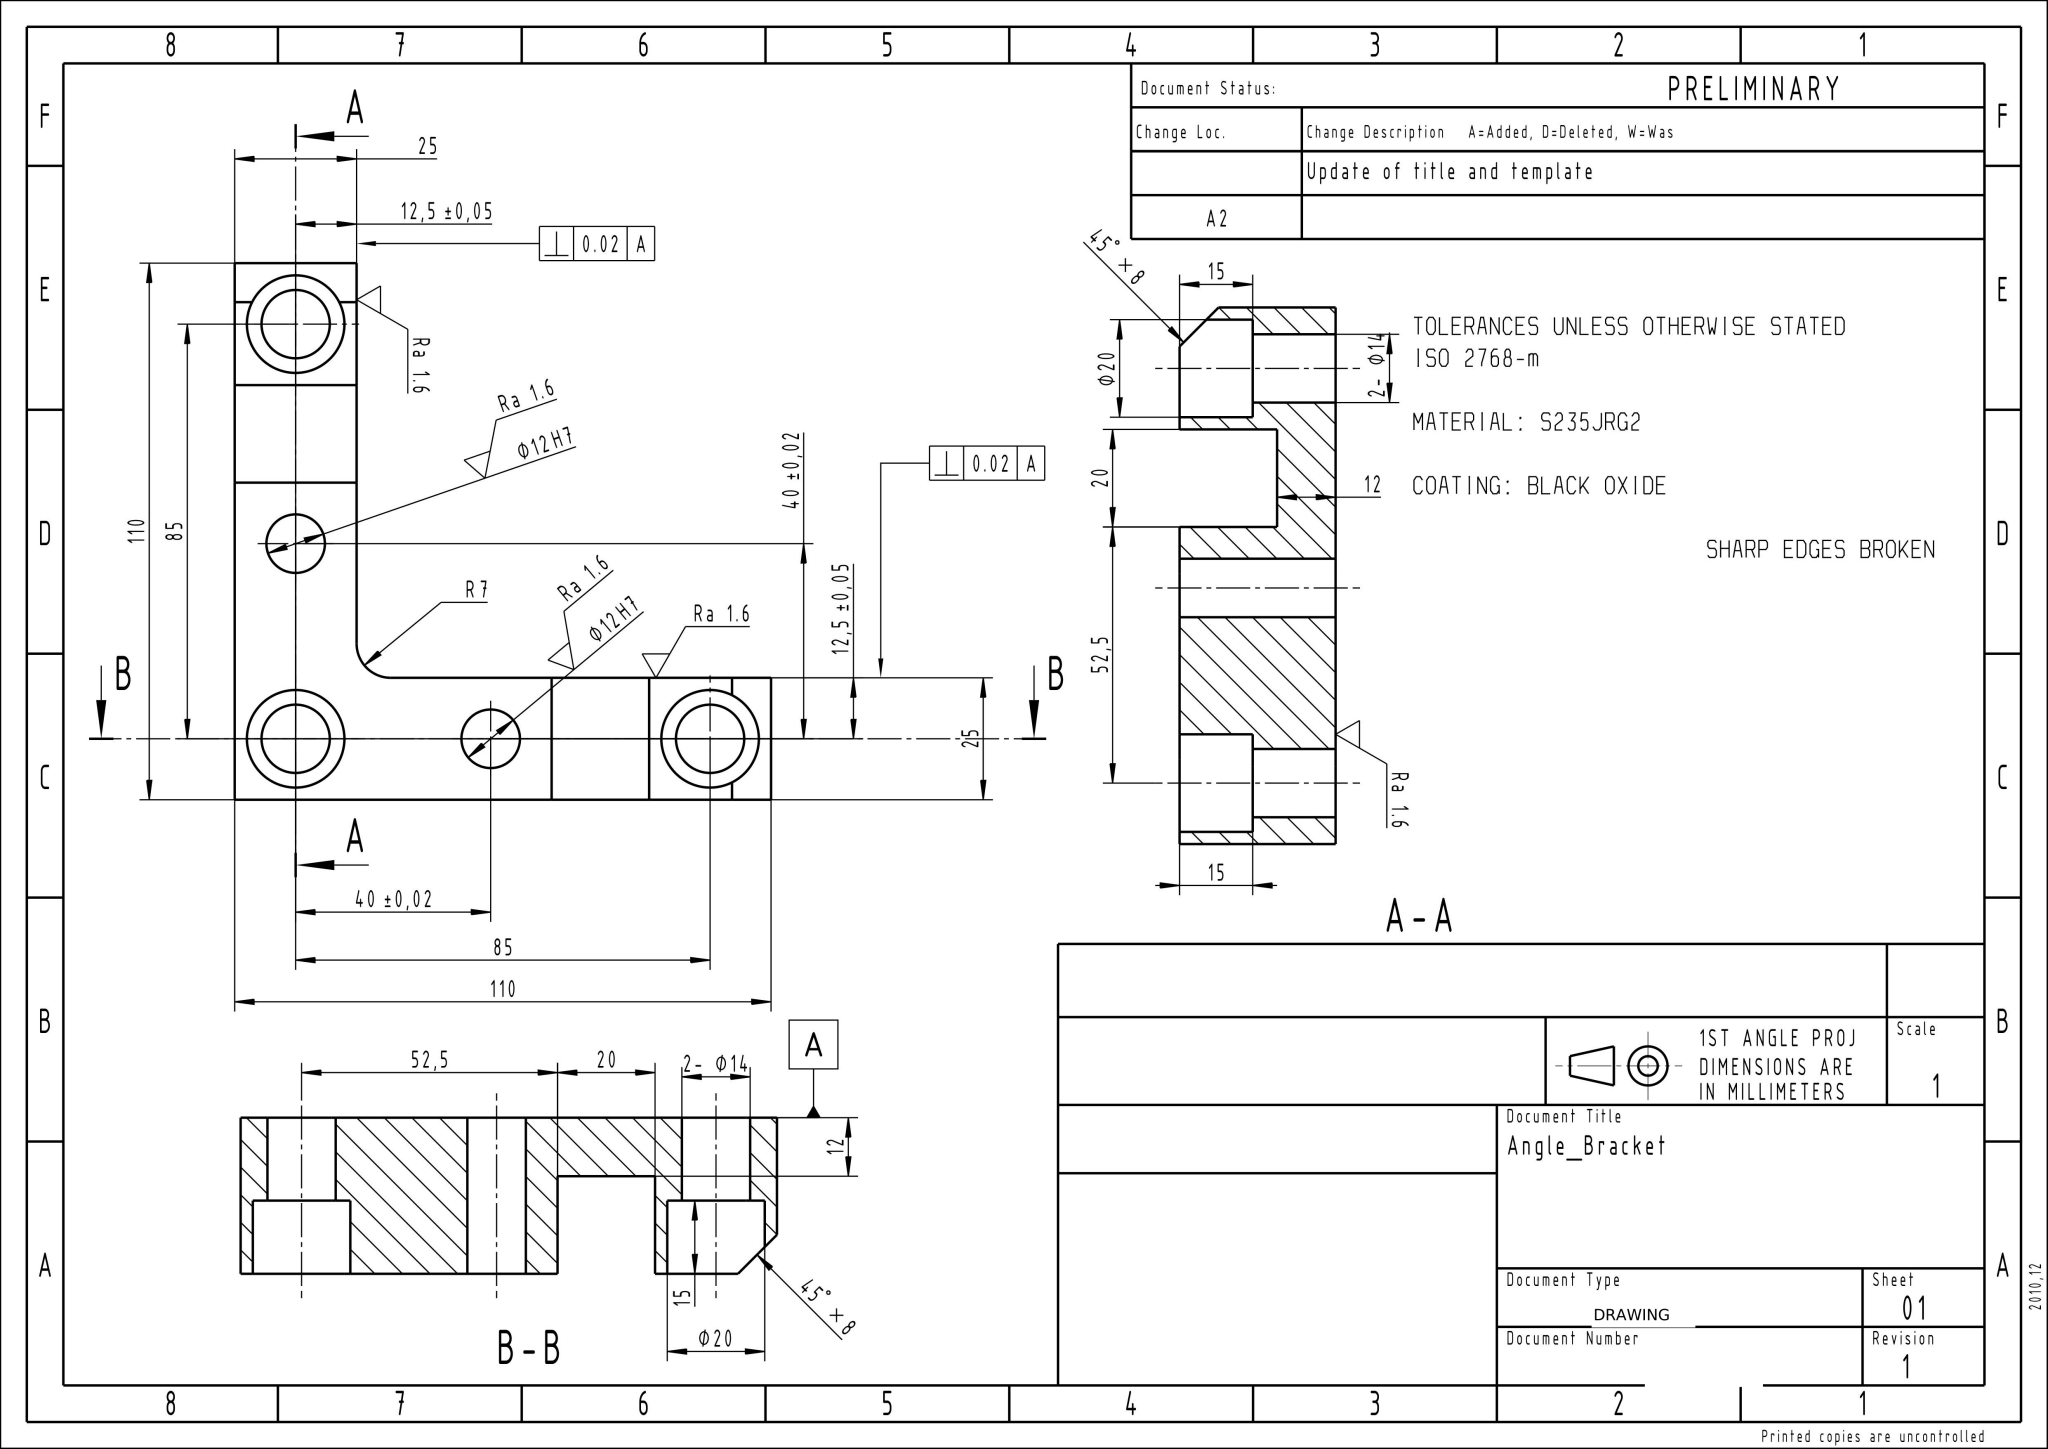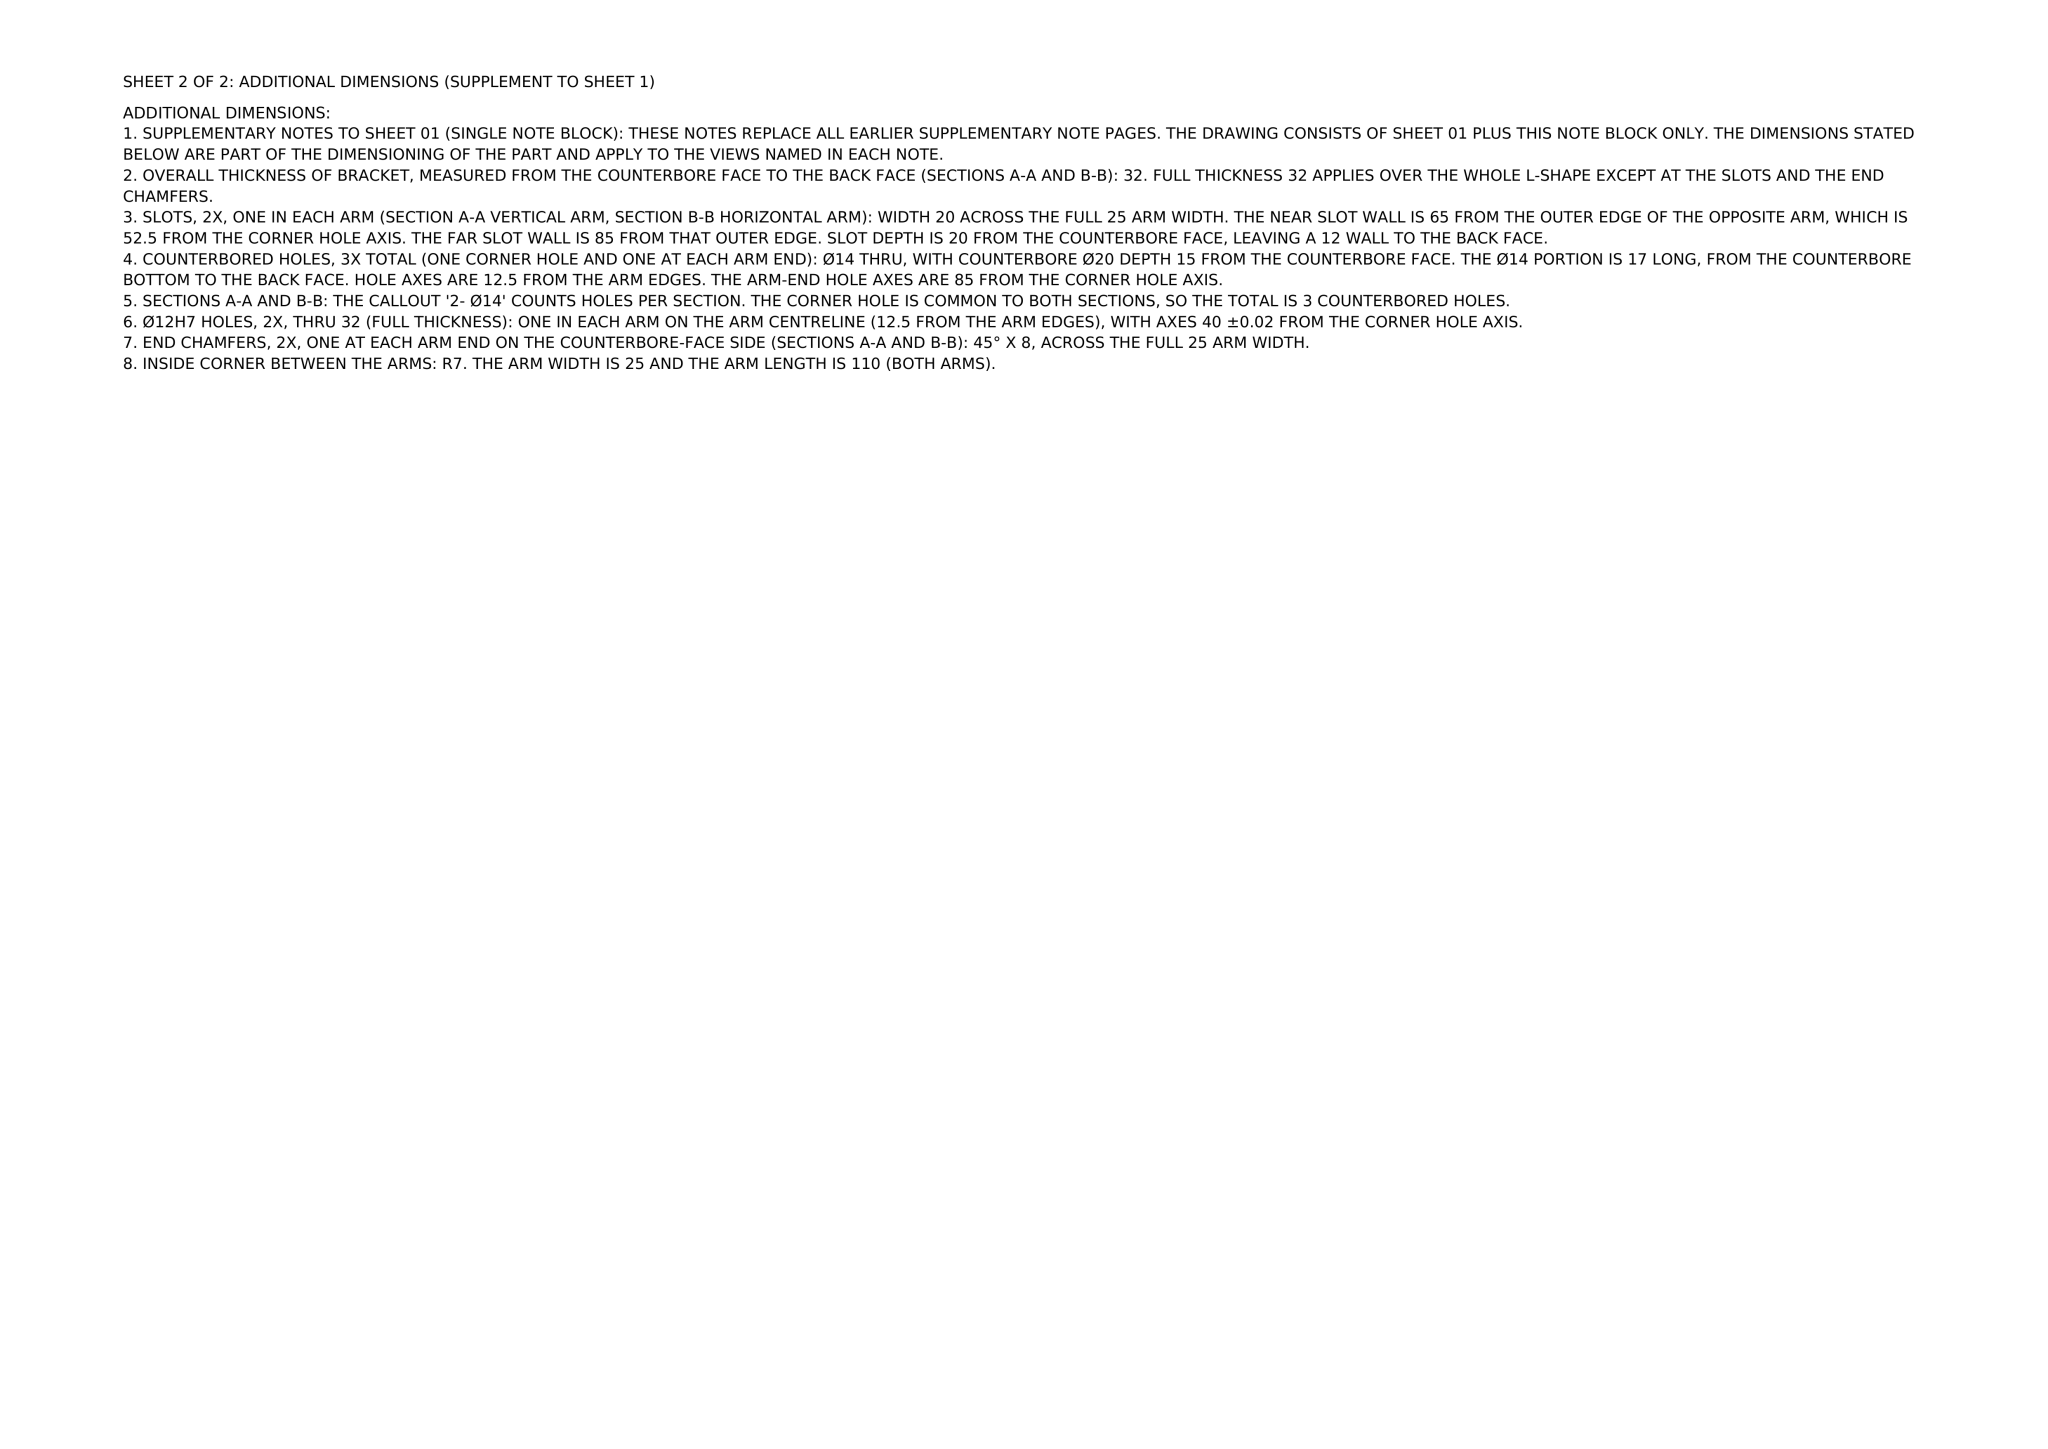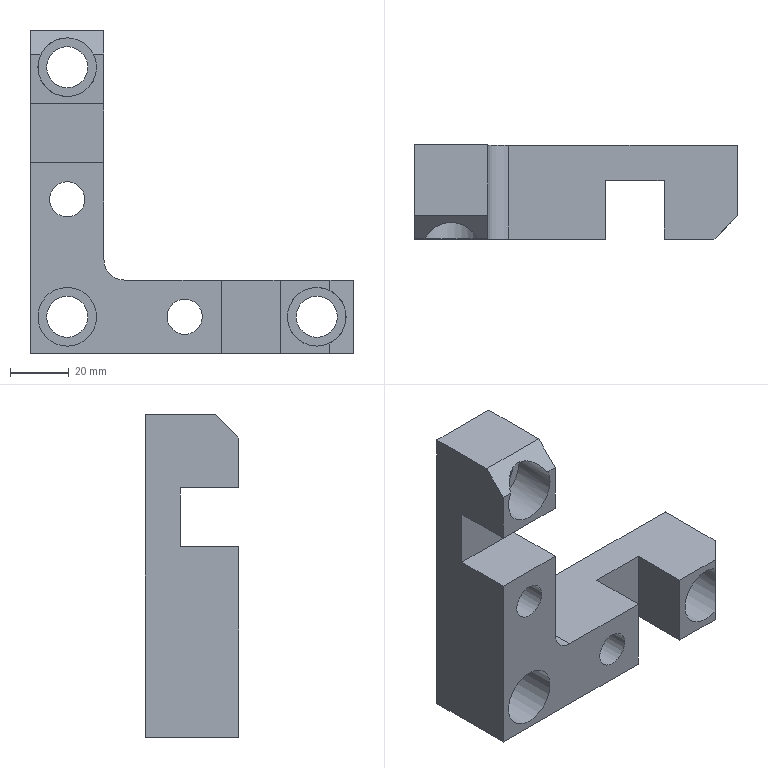Part | NX | mm | 1 solid | 30 faces | box 110 x 32 x 110 mm | volume 105828 mm3 | plane 21 | cylinder 9 | commonest cylinder face diameters 14 x4 20 x3 12 x2
STEP:
#1=CARTESIAN_POINT('',(0.,0.,0.));
#2=DIRECTION('',(0.,0.,1.));
#3=DIRECTION('',(1.,0.,0.));
#4=AXIS2_PLACEMENT_3D('',#1,#2,#3);
#5=(LENGTH_UNIT()NAMED_UNIT(*)SI_UNIT(.MILLI.,.METRE.));
#6=UNCERTAINTY_MEASURE_WITH_UNIT(LENGTH_MEASURE(0.00002),#5,'','');
#7=(NAMED_UNIT(*)PLANE_ANGLE_UNIT()SI_UNIT($,.RADIAN.));
#8=PLANE_ANGLE_MEASURE_WITH_UNIT(PLANE_ANGLE_MEASURE(0.01745),#7);
#9=DIMENSIONAL_EXPONENTS(0.,0.,0.,0.,0.,0.,0.);
#10=(CONVERSION_BASED_UNIT('',#8)NAMED_UNIT(#9)PLANE_ANGLE_UNIT());
#11=(NAMED_UNIT(*)SI_UNIT($,.STERADIAN.)SOLID_ANGLE_UNIT());
#12=(GEOMETRIC_REPRESENTATION_CONTEXT(3)GLOBAL_UNCERTAINTY_ASSIGNED_CONTEXT((#6))GLOBAL_UNIT_ASSIGNED_CONTEXT((#5,#10,#11))REPRESENTATION_CONTEXT('',''));
#13=SHAPE_REPRESENTATION('',(#4),#12);
#14=CARTESIAN_POINT('',(0.,4.,65.));
#15=VERTEX_POINT('',#14);
#16=CARTESIAN_POINT('',(25.,4.,65.));
#17=VERTEX_POINT('',#16);
#18=CARTESIAN_POINT('',(0.,4.,65.));
#19=DIRECTION('',(1.,0.,0.));
#20=VECTOR('',#19,1.);
#21=LINE('',#18,#20);
#22=EDGE_CURVE('',#15,#17,#21,.T.);
#23=ORIENTED_EDGE('',*,*,#22,.F.);
#24=CARTESIAN_POINT('',(0.,-16.,65.));
#25=VERTEX_POINT('',#24);
#26=CARTESIAN_POINT('',(0.,16.,65.));
#27=DIRECTION('',(0.,-1.,0.));
#28=VECTOR('',#27,1.);
#29=LINE('',#26,#28);
#30=EDGE_CURVE('',#15,#25,#29,.T.);
#31=ORIENTED_EDGE('',*,*,#30,.T.);
#32=CARTESIAN_POINT('',(25.,-16.,65.));
#33=VERTEX_POINT('',#32);
#34=CARTESIAN_POINT('',(0.,-16.,65.));
#35=DIRECTION('',(-1.,0.,0.));
#36=VECTOR('',#35,1.);
#37=LINE('',#34,#36);
#38=EDGE_CURVE('',#33,#25,#37,.T.);
#39=ORIENTED_EDGE('',*,*,#38,.F.);
#40=CARTESIAN_POINT('',(25.,16.,65.));
#41=DIRECTION('',(0.,-1.,0.));
#42=VECTOR('',#41,1.);
#43=LINE('',#40,#42);
#44=EDGE_CURVE('',#17,#33,#43,.T.);
#45=ORIENTED_EDGE('',*,*,#44,.F.);
#46=EDGE_LOOP('',(#23,#31,#39,#45));
#47=FACE_OUTER_BOUND('',#46,.T.);
#48=CARTESIAN_POINT('',(32.5,0.,65.));
#49=DIRECTION('',(0.,0.,-1.));
#50=DIRECTION('',(-1.,0.,0.));
#51=AXIS2_PLACEMENT_3D('',#48,#49,#50);
#52=PLANE('',#51);
#53=ADVANCED_FACE('',(#47),#52,.F.);
#54=CARTESIAN_POINT('',(12.5,-1.,19.5));
#55=VERTEX_POINT('',#54);
#56=CARTESIAN_POINT('',(12.5,-1.,12.5));
#57=DIRECTION('',(0.,-1.,0.));
#58=DIRECTION('',(0.,0.,1.));
#59=AXIS2_PLACEMENT_3D('',#56,#57,#58);
#60=CIRCLE('',#59,7.);
#61=EDGE_CURVE('',#55,#55,#60,.T.);
#62=ORIENTED_EDGE('',*,*,#61,.F.);
#63=EDGE_LOOP('',(#62));
#64=FACE_BOUND('',#63,.T.);
#65=CARTESIAN_POINT('',(12.5,-1.,22.5));
#66=VERTEX_POINT('',#65);
#67=CARTESIAN_POINT('',(12.5,-1.,12.5));
#68=DIRECTION('',(0.,-1.,0.));
#69=DIRECTION('',(0.,0.,1.));
#70=AXIS2_PLACEMENT_3D('',#67,#68,#69);
#71=CIRCLE('',#70,10.);
#72=EDGE_CURVE('',#66,#66,#71,.T.);
#73=ORIENTED_EDGE('',*,*,#72,.T.);
#74=EDGE_LOOP('',(#73));
#75=FACE_BOUND('',#74,.T.);
#76=CARTESIAN_POINT('',(12.5,-1.,12.5));
#77=DIRECTION('',(0.,1.,0.));
#78=DIRECTION('',(0.,0.,1.));
#79=AXIS2_PLACEMENT_3D('',#76,#77,#78);
#80=PLANE('',#79);
#81=ADVANCED_FACE('',(#64,#75),#80,.F.);
#82=ORIENTED_EDGE('',*,*,#72,.F.);
#83=EDGE_LOOP('',(#82));
#84=FACE_BOUND('',#83,.T.);
#85=CARTESIAN_POINT('',(12.5,-16.,22.5));
#86=VERTEX_POINT('',#85);
#87=CARTESIAN_POINT('',(12.5,-16.,12.5));
#88=DIRECTION('',(0.,1.,0.));
#89=DIRECTION('',(0.,0.,1.));
#90=AXIS2_PLACEMENT_3D('',#87,#88,#89);
#91=CIRCLE('',#90,10.);
#92=EDGE_CURVE('',#86,#86,#91,.T.);
#93=ORIENTED_EDGE('',*,*,#92,.F.);
#94=EDGE_LOOP('',(#93));
#95=FACE_BOUND('',#94,.T.);
#96=CARTESIAN_POINT('',(12.5,-16.,12.5));
#97=DIRECTION('',(0.,1.,0.));
#98=DIRECTION('',(0.,0.,1.));
#99=AXIS2_PLACEMENT_3D('',#96,#97,#98);
#100=CYLINDRICAL_SURFACE('',#99,10.);
#101=ADVANCED_FACE('',(#84,#95),#100,.F.);
#102=CARTESIAN_POINT('',(110.,16.,0.));
#103=VERTEX_POINT('',#102);
#104=CARTESIAN_POINT('',(110.,-8.,0.));
#105=VERTEX_POINT('',#104);
#106=CARTESIAN_POINT('',(110.,16.,0.));
#107=DIRECTION('',(0.,-1.,0.));
#108=VECTOR('',#107,1.);
#109=LINE('',#106,#108);
#110=EDGE_CURVE('',#103,#105,#109,.T.);
#111=ORIENTED_EDGE('',*,*,#110,.T.);
#112=CARTESIAN_POINT('',(102.,-16.,0.));
#113=VERTEX_POINT('',#112);
#114=CARTESIAN_POINT('',(67.,-51.,0.));
#115=DIRECTION('',(-0.7071,-0.7071,0.));
#116=VECTOR('',#115,1.);
#117=LINE('',#114,#116);
#118=EDGE_CURVE('',#105,#113,#117,.T.);
#119=ORIENTED_EDGE('',*,*,#118,.T.);
#120=CARTESIAN_POINT('',(85.,-16.,0.));
#121=VERTEX_POINT('',#120);
#122=CARTESIAN_POINT('',(0.,-16.,0.));
#123=DIRECTION('',(1.,0.,0.));
#124=VECTOR('',#123,1.);
#125=LINE('',#122,#124);
#126=EDGE_CURVE('',#121,#113,#125,.T.);
#127=ORIENTED_EDGE('',*,*,#126,.F.);
#128=CARTESIAN_POINT('',(85.,4.,0.));
#129=VERTEX_POINT('',#128);
#130=CARTESIAN_POINT('',(85.,16.,0.));
#131=DIRECTION('',(0.,-1.,0.));
#132=VECTOR('',#131,1.);
#133=LINE('',#130,#132);
#134=EDGE_CURVE('',#129,#121,#133,.T.);
#135=ORIENTED_EDGE('',*,*,#134,.F.);
#136=CARTESIAN_POINT('',(65.,4.,0.));
#137=VERTEX_POINT('',#136);
#138=CARTESIAN_POINT('',(0.,4.,0.));
#139=DIRECTION('',(1.,0.,0.));
#140=VECTOR('',#139,1.);
#141=LINE('',#138,#140);
#142=EDGE_CURVE('',#137,#129,#141,.T.);
#143=ORIENTED_EDGE('',*,*,#142,.F.);
#144=CARTESIAN_POINT('',(65.,-16.,0.));
#145=VERTEX_POINT('',#144);
#146=CARTESIAN_POINT('',(65.,16.,0.));
#147=DIRECTION('',(0.,1.,0.));
#148=VECTOR('',#147,1.);
#149=LINE('',#146,#148);
#150=EDGE_CURVE('',#145,#137,#149,.T.);
#151=ORIENTED_EDGE('',*,*,#150,.F.);
#152=CARTESIAN_POINT('',(0.,-16.,0.));
#153=VERTEX_POINT('',#152);
#154=CARTESIAN_POINT('',(0.,-16.,0.));
#155=DIRECTION('',(1.,0.,0.));
#156=VECTOR('',#155,1.);
#157=LINE('',#154,#156);
#158=EDGE_CURVE('',#153,#145,#157,.T.);
#159=ORIENTED_EDGE('',*,*,#158,.F.);
#160=CARTESIAN_POINT('',(0.,16.,0.));
#161=VERTEX_POINT('',#160);
#162=CARTESIAN_POINT('',(0.,16.,0.));
#163=DIRECTION('',(0.,-1.,0.));
#164=VECTOR('',#163,1.);
#165=LINE('',#162,#164);
#166=EDGE_CURVE('',#161,#153,#165,.T.);
#167=ORIENTED_EDGE('',*,*,#166,.F.);
#168=CARTESIAN_POINT('',(0.,16.,0.));
#169=DIRECTION('',(1.,0.,0.));
#170=VECTOR('',#169,1.);
#171=LINE('',#168,#170);
#172=EDGE_CURVE('',#161,#103,#171,.T.);
#173=ORIENTED_EDGE('',*,*,#172,.T.);
#174=EDGE_LOOP('',(#111,#119,#127,#135,#143,#151,#159,#167,#173));
#175=FACE_OUTER_BOUND('',#174,.T.);
#176=CARTESIAN_POINT('',(0.,16.,0.));
#177=DIRECTION('',(0.,0.,-1.));
#178=DIRECTION('',(-1.,0.,0.));
#179=AXIS2_PLACEMENT_3D('',#176,#177,#178);
#180=PLANE('',#179);
#181=ADVANCED_FACE('',(#175),#180,.T.);
#182=ORIENTED_EDGE('',*,*,#150,.T.);
#183=CARTESIAN_POINT('',(65.,4.,25.));
#184=VERTEX_POINT('',#183);
#185=CARTESIAN_POINT('',(65.,4.,110.));
#186=DIRECTION('',(0.,0.,1.));
#187=VECTOR('',#186,1.);
#188=LINE('',#185,#187);
#189=EDGE_CURVE('',#137,#184,#188,.T.);
#190=ORIENTED_EDGE('',*,*,#189,.T.);
#191=CARTESIAN_POINT('',(65.,-16.,25.));
#192=VERTEX_POINT('',#191);
#193=CARTESIAN_POINT('',(65.,16.,25.));
#194=DIRECTION('',(0.,1.,0.));
#195=VECTOR('',#194,1.);
#196=LINE('',#193,#195);
#197=EDGE_CURVE('',#192,#184,#196,.T.);
#198=ORIENTED_EDGE('',*,*,#197,.F.);
#199=CARTESIAN_POINT('',(65.,-16.,110.));
#200=DIRECTION('',(0.,0.,-1.));
#201=VECTOR('',#200,1.);
#202=LINE('',#199,#201);
#203=EDGE_CURVE('',#192,#145,#202,.T.);
#204=ORIENTED_EDGE('',*,*,#203,.T.);
#205=EDGE_LOOP('',(#182,#190,#198,#204));
#206=FACE_OUTER_BOUND('',#205,.T.);
#207=CARTESIAN_POINT('',(65.,0.,55.));
#208=DIRECTION('',(-1.,0.,0.));
#209=DIRECTION('',(0.,0.,1.));
#210=AXIS2_PLACEMENT_3D('',#207,#208,#209);
#211=PLANE('',#210);
#212=ADVANCED_FACE('',(#206),#211,.F.);
#213=CARTESIAN_POINT('',(32.,16.,25.));
#214=VERTEX_POINT('',#213);
#215=CARTESIAN_POINT('',(110.,16.,25.));
#216=VERTEX_POINT('',#215);
#217=CARTESIAN_POINT('',(0.,16.,25.));
#218=DIRECTION('',(1.,0.,0.));
#219=VECTOR('',#218,1.);
#220=LINE('',#217,#219);
#221=EDGE_CURVE('',#214,#216,#220,.T.);
#222=ORIENTED_EDGE('',*,*,#221,.F.);
#223=CARTESIAN_POINT('',(32.,-16.,25.));
#224=VERTEX_POINT('',#223);
#225=CARTESIAN_POINT('',(32.,-16.,25.));
#226=DIRECTION('',(0.,-1.,0.));
#227=VECTOR('',#226,1.);
#228=LINE('',#225,#227);
#229=EDGE_CURVE('',#214,#224,#228,.T.);
#230=ORIENTED_EDGE('',*,*,#229,.T.);
#231=CARTESIAN_POINT('',(0.,-16.,25.));
#232=DIRECTION('',(1.,0.,0.));
#233=VECTOR('',#232,1.);
#234=LINE('',#231,#233);
#235=EDGE_CURVE('',#224,#192,#234,.T.);
#236=ORIENTED_EDGE('',*,*,#235,.T.);
#237=ORIENTED_EDGE('',*,*,#197,.T.);
#238=CARTESIAN_POINT('',(85.,4.,25.));
#239=VERTEX_POINT('',#238);
#240=CARTESIAN_POINT('',(0.,4.,25.));
#241=DIRECTION('',(1.,0.,0.));
#242=VECTOR('',#241,1.);
#243=LINE('',#240,#242);
#244=EDGE_CURVE('',#184,#239,#243,.T.);
#245=ORIENTED_EDGE('',*,*,#244,.T.);
#246=CARTESIAN_POINT('',(85.,-16.,25.));
#247=VERTEX_POINT('',#246);
#248=CARTESIAN_POINT('',(85.,16.,25.));
#249=DIRECTION('',(0.,1.,0.));
#250=VECTOR('',#249,1.);
#251=LINE('',#248,#250);
#252=EDGE_CURVE('',#247,#239,#251,.T.);
#253=ORIENTED_EDGE('',*,*,#252,.F.);
#254=CARTESIAN_POINT('',(102.,-16.,25.));
#255=VERTEX_POINT('',#254);
#256=CARTESIAN_POINT('',(0.,-16.,25.));
#257=DIRECTION('',(1.,0.,0.));
#258=VECTOR('',#257,1.);
#259=LINE('',#256,#258);
#260=EDGE_CURVE('',#247,#255,#259,.T.);
#261=ORIENTED_EDGE('',*,*,#260,.T.);
#262=CARTESIAN_POINT('',(110.,-8.,25.));
#263=VERTEX_POINT('',#262);
#264=CARTESIAN_POINT('',(102.,-16.,25.));
#265=DIRECTION('',(0.7071,0.7071,0.));
#266=VECTOR('',#265,1.);
#267=LINE('',#264,#266);
#268=EDGE_CURVE('',#255,#263,#267,.T.);
#269=ORIENTED_EDGE('',*,*,#268,.T.);
#270=CARTESIAN_POINT('',(110.,16.,25.));
#271=DIRECTION('',(0.,-1.,0.));
#272=VECTOR('',#271,1.);
#273=LINE('',#270,#272);
#274=EDGE_CURVE('',#216,#263,#273,.T.);
#275=ORIENTED_EDGE('',*,*,#274,.F.);
#276=EDGE_LOOP('',(#222,#230,#236,#237,#245,#253,#261,#269,#275));
#277=FACE_OUTER_BOUND('',#276,.T.);
#278=CARTESIAN_POINT('',(0.,16.,25.));
#279=DIRECTION('',(0.,0.,-1.));
#280=DIRECTION('',(-1.,0.,0.));
#281=AXIS2_PLACEMENT_3D('',#278,#279,#280);
#282=PLANE('',#281);
#283=ADVANCED_FACE('',(#277),#282,.F.);
#284=ORIENTED_EDGE('',*,*,#61,.T.);
#285=EDGE_LOOP('',(#284));
#286=FACE_BOUND('',#285,.T.);
#287=CARTESIAN_POINT('',(12.5,16.,19.5));
#288=VERTEX_POINT('',#287);
#289=CARTESIAN_POINT('',(12.5,16.,12.5));
#290=DIRECTION('',(0.,-1.,0.));
#291=DIRECTION('',(0.,0.,1.));
#292=AXIS2_PLACEMENT_3D('',#289,#290,#291);
#293=CIRCLE('',#292,7.);
#294=EDGE_CURVE('',#288,#288,#293,.T.);
#295=ORIENTED_EDGE('',*,*,#294,.F.);
#296=EDGE_LOOP('',(#295));
#297=FACE_BOUND('',#296,.T.);
#298=CARTESIAN_POINT('',(12.5,63.386,12.5));
#299=DIRECTION('',(0.,1.,0.));
#300=DIRECTION('',(0.,0.,1.));
#301=AXIS2_PLACEMENT_3D('',#298,#299,#300);
#302=CYLINDRICAL_SURFACE('',#301,7.);
#303=ADVANCED_FACE('',(#286,#297),#302,.F.);
#304=CARTESIAN_POINT('',(12.5,-16.,58.5));
#305=VERTEX_POINT('',#304);
#306=CARTESIAN_POINT('',(12.5,-16.,52.5));
#307=DIRECTION('',(0.,1.,0.));
#308=DIRECTION('',(0.,0.,1.));
#309=AXIS2_PLACEMENT_3D('',#306,#307,#308);
#310=CIRCLE('',#309,6.);
#311=EDGE_CURVE('',#305,#305,#310,.T.);
#312=ORIENTED_EDGE('',*,*,#311,.F.);
#313=EDGE_LOOP('',(#312));
#314=FACE_BOUND('',#313,.T.);
#315=CARTESIAN_POINT('',(12.5,16.,58.5));
#316=VERTEX_POINT('',#315);
#317=CARTESIAN_POINT('',(12.5,16.,52.5));
#318=DIRECTION('',(0.,-1.,0.));
#319=DIRECTION('',(0.,0.,1.));
#320=AXIS2_PLACEMENT_3D('',#317,#318,#319);
#321=CIRCLE('',#320,6.);
#322=EDGE_CURVE('',#316,#316,#321,.T.);
#323=ORIENTED_EDGE('',*,*,#322,.F.);
#324=EDGE_LOOP('',(#323));
#325=FACE_BOUND('',#324,.T.);
#326=CARTESIAN_POINT('',(12.5,-16.,52.5));
#327=DIRECTION('',(0.,1.,0.));
#328=DIRECTION('',(0.,0.,1.));
#329=AXIS2_PLACEMENT_3D('',#326,#327,#328);
#330=CYLINDRICAL_SURFACE('',#329,6.);
#331=ADVANCED_FACE('',(#314,#325),#330,.F.);
#332=CARTESIAN_POINT('',(52.5,-16.,18.5));
#333=VERTEX_POINT('',#332);
#334=CARTESIAN_POINT('',(52.5,-16.,12.5));
#335=DIRECTION('',(0.,1.,0.));
#336=DIRECTION('',(0.,0.,1.));
#337=AXIS2_PLACEMENT_3D('',#334,#335,#336);
#338=CIRCLE('',#337,6.);
#339=EDGE_CURVE('',#333,#333,#338,.T.);
#340=ORIENTED_EDGE('',*,*,#339,.F.);
#341=EDGE_LOOP('',(#340));
#342=FACE_BOUND('',#341,.T.);
#343=CARTESIAN_POINT('',(52.5,16.,18.5));
#344=VERTEX_POINT('',#343);
#345=CARTESIAN_POINT('',(52.5,16.,12.5));
#346=DIRECTION('',(0.,-1.,0.));
#347=DIRECTION('',(0.,0.,1.));
#348=AXIS2_PLACEMENT_3D('',#345,#346,#347);
#349=CIRCLE('',#348,6.);
#350=EDGE_CURVE('',#344,#344,#349,.T.);
#351=ORIENTED_EDGE('',*,*,#350,.F.);
#352=EDGE_LOOP('',(#351));
#353=FACE_BOUND('',#352,.T.);
#354=CARTESIAN_POINT('',(52.5,-16.,12.5));
#355=DIRECTION('',(0.,1.,0.));
#356=DIRECTION('',(0.,0.,1.));
#357=AXIS2_PLACEMENT_3D('',#354,#355,#356);
#358=CYLINDRICAL_SURFACE('',#357,6.);
#359=ADVANCED_FACE('',(#342,#353),#358,.F.);
#360=ORIENTED_EDGE('',*,*,#339,.T.);
#361=EDGE_LOOP('',(#360));
#362=FACE_BOUND('',#361,.T.);
#363=ORIENTED_EDGE('',*,*,#311,.T.);
#364=EDGE_LOOP('',(#363));
#365=FACE_BOUND('',#364,.T.);
#366=ORIENTED_EDGE('',*,*,#92,.T.);
#367=EDGE_LOOP('',(#366));
#368=FACE_BOUND('',#367,.T.);
#369=CARTESIAN_POINT('',(25.,-16.,32.));
#370=VERTEX_POINT('',#369);
#371=CARTESIAN_POINT('',(25.,-16.,110.));
#372=DIRECTION('',(0.,0.,-1.));
#373=VECTOR('',#372,1.);
#374=LINE('',#371,#373);
#375=EDGE_CURVE('',#33,#370,#374,.T.);
#376=ORIENTED_EDGE('',*,*,#375,.F.);
#377=ORIENTED_EDGE('',*,*,#38,.T.);
#378=CARTESIAN_POINT('',(0.,-16.,110.));
#379=DIRECTION('',(0.,0.,-1.));
#380=VECTOR('',#379,1.);
#381=LINE('',#378,#380);
#382=EDGE_CURVE('',#25,#153,#381,.T.);
#383=ORIENTED_EDGE('',*,*,#382,.T.);
#384=ORIENTED_EDGE('',*,*,#158,.T.);
#385=ORIENTED_EDGE('',*,*,#203,.F.);
#386=ORIENTED_EDGE('',*,*,#235,.F.);
#387=CARTESIAN_POINT('',(32.,-16.,32.));
#388=DIRECTION('',(0.,1.,0.));
#389=DIRECTION('',(0.,0.,1.));
#390=AXIS2_PLACEMENT_3D('',#387,#388,#389);
#391=CIRCLE('',#390,7.);
#392=EDGE_CURVE('',#224,#370,#391,.T.);
#393=ORIENTED_EDGE('',*,*,#392,.T.);
#394=EDGE_LOOP('',(#376,#377,#383,#384,#385,#386,#393));
#395=FACE_BOUND('',#394,.T.);
#396=CARTESIAN_POINT('',(0.,-16.,110.));
#397=DIRECTION('',(0.,1.,0.));
#398=DIRECTION('',(0.,0.,-1.));
#399=AXIS2_PLACEMENT_3D('',#396,#397,#398);
#400=PLANE('',#399);
#401=ADVANCED_FACE('',(#362,#365,#368,#395),#400,.F.);
#402=ORIENTED_EDGE('',*,*,#350,.T.);
#403=EDGE_LOOP('',(#402));
#404=FACE_BOUND('',#403,.T.);
#405=ORIENTED_EDGE('',*,*,#322,.T.);
#406=EDGE_LOOP('',(#405));
#407=FACE_BOUND('',#406,.T.);
#408=ORIENTED_EDGE('',*,*,#294,.T.);
#409=EDGE_LOOP('',(#408));
#410=FACE_BOUND('',#409,.T.);
#411=CARTESIAN_POINT('',(0.,16.,110.));
#412=VERTEX_POINT('',#411);
#413=CARTESIAN_POINT('',(0.,16.,110.));
#414=DIRECTION('',(0.,0.,-1.));
#415=VECTOR('',#414,1.);
#416=LINE('',#413,#415);
#417=EDGE_CURVE('',#412,#161,#416,.T.);
#418=ORIENTED_EDGE('',*,*,#417,.F.);
#419=CARTESIAN_POINT('',(25.,16.,110.));
#420=VERTEX_POINT('',#419);
#421=CARTESIAN_POINT('',(0.,16.,110.));
#422=DIRECTION('',(1.,0.,0.));
#423=VECTOR('',#422,1.);
#424=LINE('',#421,#423);
#425=EDGE_CURVE('',#412,#420,#424,.T.);
#426=ORIENTED_EDGE('',*,*,#425,.T.);
#427=CARTESIAN_POINT('',(25.,16.,32.));
#428=VERTEX_POINT('',#427);
#429=CARTESIAN_POINT('',(25.,16.,110.));
#430=DIRECTION('',(0.,0.,-1.));
#431=VECTOR('',#430,1.);
#432=LINE('',#429,#431);
#433=EDGE_CURVE('',#420,#428,#432,.T.);
#434=ORIENTED_EDGE('',*,*,#433,.T.);
#435=CARTESIAN_POINT('',(32.,16.,32.));
#436=DIRECTION('',(0.,-1.,0.));
#437=DIRECTION('',(0.,0.,1.));
#438=AXIS2_PLACEMENT_3D('',#435,#436,#437);
#439=CIRCLE('',#438,7.);
#440=EDGE_CURVE('',#428,#214,#439,.T.);
#441=ORIENTED_EDGE('',*,*,#440,.T.);
#442=ORIENTED_EDGE('',*,*,#221,.T.);
#443=CARTESIAN_POINT('',(110.,16.,0.));
#444=DIRECTION('',(0.,0.,1.));
#445=VECTOR('',#444,1.);
#446=LINE('',#443,#445);
#447=EDGE_CURVE('',#103,#216,#446,.T.);
#448=ORIENTED_EDGE('',*,*,#447,.F.);
#449=ORIENTED_EDGE('',*,*,#172,.F.);
#450=EDGE_LOOP('',(#418,#426,#434,#441,#442,#448,#449));
#451=FACE_BOUND('',#450,.T.);
#452=CARTESIAN_POINT('',(12.5,16.,104.5));
#453=VERTEX_POINT('',#452);
#454=CARTESIAN_POINT('',(12.5,16.,97.5));
#455=DIRECTION('',(0.,-1.,0.));
#456=DIRECTION('',(0.,0.,1.));
#457=AXIS2_PLACEMENT_3D('',#454,#455,#456);
#458=CIRCLE('',#457,7.);
#459=EDGE_CURVE('',#453,#453,#458,.T.);
#460=ORIENTED_EDGE('',*,*,#459,.T.);
#461=EDGE_LOOP('',(#460));
#462=FACE_BOUND('',#461,.T.);
#463=CARTESIAN_POINT('',(97.5,16.,19.5));
#464=VERTEX_POINT('',#463);
#465=CARTESIAN_POINT('',(97.5,16.,12.5));
#466=DIRECTION('',(0.,-1.,0.));
#467=DIRECTION('',(0.,0.,1.));
#468=AXIS2_PLACEMENT_3D('',#465,#466,#467);
#469=CIRCLE('',#468,7.);
#470=EDGE_CURVE('',#464,#464,#469,.T.);
#471=ORIENTED_EDGE('',*,*,#470,.T.);
#472=EDGE_LOOP('',(#471));
#473=FACE_BOUND('',#472,.T.);
#474=CARTESIAN_POINT('',(0.,16.,0.));
#475=DIRECTION('',(0.,1.,0.));
#476=DIRECTION('',(1.,0.,0.));
#477=AXIS2_PLACEMENT_3D('',#474,#475,#476);
#478=PLANE('',#477);
#479=ADVANCED_FACE('',(#404,#407,#410,#451,#462,#473),#478,.T.);
#480=CARTESIAN_POINT('',(0.,-16.,102.));
#481=VERTEX_POINT('',#480);
#482=CARTESIAN_POINT('',(0.,-16.,85.));
#483=VERTEX_POINT('',#482);
#484=CARTESIAN_POINT('',(0.,-16.,110.));
#485=DIRECTION('',(0.,0.,-1.));
#486=VECTOR('',#485,1.);
#487=LINE('',#484,#486);
#488=EDGE_CURVE('',#481,#483,#487,.T.);
#489=ORIENTED_EDGE('',*,*,#488,.F.);
#490=CARTESIAN_POINT('',(0.,-8.,110.));
#491=VERTEX_POINT('',#490);
#492=CARTESIAN_POINT('',(0.,4.,122.));
#493=DIRECTION('',(0.,0.7071,0.7071));
#494=VECTOR('',#493,1.);
#495=LINE('',#492,#494);
#496=EDGE_CURVE('',#481,#491,#495,.T.);
#497=ORIENTED_EDGE('',*,*,#496,.T.);
#498=CARTESIAN_POINT('',(0.,16.,110.));
#499=DIRECTION('',(0.,-1.,0.));
#500=VECTOR('',#499,1.);
#501=LINE('',#498,#500);
#502=EDGE_CURVE('',#412,#491,#501,.T.);
#503=ORIENTED_EDGE('',*,*,#502,.F.);
#504=ORIENTED_EDGE('',*,*,#417,.T.);
#505=ORIENTED_EDGE('',*,*,#166,.T.);
#506=ORIENTED_EDGE('',*,*,#382,.F.);
#507=ORIENTED_EDGE('',*,*,#30,.F.);
#508=CARTESIAN_POINT('',(0.,4.,85.));
#509=VERTEX_POINT('',#508);
#510=CARTESIAN_POINT('',(0.,4.,110.));
#511=DIRECTION('',(0.,0.,-1.));
#512=VECTOR('',#511,1.);
#513=LINE('',#510,#512);
#514=EDGE_CURVE('',#509,#15,#513,.T.);
#515=ORIENTED_EDGE('',*,*,#514,.F.);
#516=CARTESIAN_POINT('',(0.,16.,85.));
#517=DIRECTION('',(0.,1.,0.));
#518=VECTOR('',#517,1.);
#519=LINE('',#516,#518);
#520=EDGE_CURVE('',#483,#509,#519,.T.);
#521=ORIENTED_EDGE('',*,*,#520,.F.);
#522=EDGE_LOOP('',(#489,#497,#503,#504,#505,#506,#507,#515,#521));
#523=FACE_OUTER_BOUND('',#522,.T.);
#524=CARTESIAN_POINT('',(0.,16.,110.));
#525=DIRECTION('',(-1.,0.,0.));
#526=DIRECTION('',(0.,0.,1.));
#527=AXIS2_PLACEMENT_3D('',#524,#525,#526);
#528=PLANE('',#527);
#529=ADVANCED_FACE('',(#523),#528,.T.);
#530=ORIENTED_EDGE('',*,*,#375,.T.);
#531=CARTESIAN_POINT('',(25.,16.,32.));
#532=DIRECTION('',(0.,1.,0.));
#533=VECTOR('',#532,1.);
#534=LINE('',#531,#533);
#535=EDGE_CURVE('',#370,#428,#534,.T.);
#536=ORIENTED_EDGE('',*,*,#535,.T.);
#537=ORIENTED_EDGE('',*,*,#433,.F.);
#538=CARTESIAN_POINT('',(25.,-8.,110.));
#539=VERTEX_POINT('',#538);
#540=CARTESIAN_POINT('',(25.,16.,110.));
#541=DIRECTION('',(0.,-1.,0.));
#542=VECTOR('',#541,1.);
#543=LINE('',#540,#542);
#544=EDGE_CURVE('',#420,#539,#543,.T.);
#545=ORIENTED_EDGE('',*,*,#544,.T.);
#546=CARTESIAN_POINT('',(25.,-16.,102.));
#547=VERTEX_POINT('',#546);
#548=CARTESIAN_POINT('',(25.,-8.,110.));
#549=DIRECTION('',(0.,-0.7071,-0.7071));
#550=VECTOR('',#549,1.);
#551=LINE('',#548,#550);
#552=EDGE_CURVE('',#539,#547,#551,.T.);
#553=ORIENTED_EDGE('',*,*,#552,.T.);
#554=CARTESIAN_POINT('',(25.,-16.,85.));
#555=VERTEX_POINT('',#554);
#556=CARTESIAN_POINT('',(25.,-16.,110.));
#557=DIRECTION('',(0.,0.,-1.));
#558=VECTOR('',#557,1.);
#559=LINE('',#556,#558);
#560=EDGE_CURVE('',#547,#555,#559,.T.);
#561=ORIENTED_EDGE('',*,*,#560,.T.);
#562=CARTESIAN_POINT('',(25.,4.,85.));
#563=VERTEX_POINT('',#562);
#564=CARTESIAN_POINT('',(25.,16.,85.));
#565=DIRECTION('',(0.,1.,0.));
#566=VECTOR('',#565,1.);
#567=LINE('',#564,#566);
#568=EDGE_CURVE('',#555,#563,#567,.T.);
#569=ORIENTED_EDGE('',*,*,#568,.T.);
#570=CARTESIAN_POINT('',(25.,4.,110.));
#571=DIRECTION('',(0.,0.,-1.));
#572=VECTOR('',#571,1.);
#573=LINE('',#570,#572);
#574=EDGE_CURVE('',#563,#17,#573,.T.);
#575=ORIENTED_EDGE('',*,*,#574,.T.);
#576=ORIENTED_EDGE('',*,*,#44,.T.);
#577=EDGE_LOOP('',(#530,#536,#537,#545,#553,#561,#569,#575,#576));
#578=FACE_OUTER_BOUND('',#577,.T.);
#579=CARTESIAN_POINT('',(25.,16.,110.));
#580=DIRECTION('',(-1.,0.,0.));
#581=DIRECTION('',(0.,0.,1.));
#582=AXIS2_PLACEMENT_3D('',#579,#580,#581);
#583=PLANE('',#582);
#584=ADVANCED_FACE('',(#578),#583,.F.);
#585=ORIENTED_EDGE('',*,*,#520,.T.);
#586=CARTESIAN_POINT('',(0.,4.,85.));
#587=DIRECTION('',(1.,0.,0.));
#588=VECTOR('',#587,1.);
#589=LINE('',#586,#588);
#590=EDGE_CURVE('',#509,#563,#589,.T.);
#591=ORIENTED_EDGE('',*,*,#590,.T.);
#592=ORIENTED_EDGE('',*,*,#568,.F.);
#593=CARTESIAN_POINT('',(0.,-16.,85.));
#594=DIRECTION('',(-1.,0.,0.));
#595=VECTOR('',#594,1.);
#596=LINE('',#593,#595);
#597=EDGE_CURVE('',#555,#483,#596,.T.);
#598=ORIENTED_EDGE('',*,*,#597,.T.);
#599=EDGE_LOOP('',(#585,#591,#592,#598));
#600=FACE_OUTER_BOUND('',#599,.T.);
#601=CARTESIAN_POINT('',(12.5,0.,85.));
#602=DIRECTION('',(0.,0.,-1.));
#603=DIRECTION('',(-1.,0.,0.));
#604=AXIS2_PLACEMENT_3D('',#601,#602,#603);
#605=PLANE('',#604);
#606=ADVANCED_FACE('',(#600),#605,.T.);
#607=ORIENTED_EDGE('',*,*,#560,.F.);
#608=CARTESIAN_POINT('',(21.43,-16.,102.));
#609=VERTEX_POINT('',#608);
#610=CARTESIAN_POINT('',(0.,-16.,102.));
#611=DIRECTION('',(-1.,0.,0.));
#612=VECTOR('',#611,1.);
#613=LINE('',#610,#612);
#614=EDGE_CURVE('',#547,#609,#613,.T.);
#615=ORIENTED_EDGE('',*,*,#614,.T.);
#616=CARTESIAN_POINT('',(3.57,-16.,102.));
#617=VERTEX_POINT('',#616);
#618=CARTESIAN_POINT('',(12.5,-16.,97.5));
#619=DIRECTION('',(0.,1.,0.));
#620=DIRECTION('',(0.,0.,1.));
#621=AXIS2_PLACEMENT_3D('',#618,#619,#620);
#622=CIRCLE('',#621,10.);
#623=EDGE_CURVE('',#609,#617,#622,.T.);
#624=ORIENTED_EDGE('',*,*,#623,.T.);
#625=CARTESIAN_POINT('',(0.,-16.,102.));
#626=DIRECTION('',(-1.,0.,0.));
#627=VECTOR('',#626,1.);
#628=LINE('',#625,#627);
#629=EDGE_CURVE('',#617,#481,#628,.T.);
#630=ORIENTED_EDGE('',*,*,#629,.T.);
#631=ORIENTED_EDGE('',*,*,#488,.T.);
#632=ORIENTED_EDGE('',*,*,#597,.F.);
#633=EDGE_LOOP('',(#607,#615,#624,#630,#631,#632));
#634=FACE_OUTER_BOUND('',#633,.T.);
#635=CARTESIAN_POINT('',(0.,-16.,110.));
#636=DIRECTION('',(0.,1.,0.));
#637=DIRECTION('',(0.,0.,-1.));
#638=AXIS2_PLACEMENT_3D('',#635,#636,#637);
#639=PLANE('',#638);
#640=ADVANCED_FACE('',(#634),#639,.F.);
#641=CARTESIAN_POINT('',(12.5,-1.,104.5));
#642=VERTEX_POINT('',#641);
#643=CARTESIAN_POINT('',(12.5,-1.,97.5));
#644=DIRECTION('',(0.,-1.,0.));
#645=DIRECTION('',(0.,0.,1.));
#646=AXIS2_PLACEMENT_3D('',#643,#644,#645);
#647=CIRCLE('',#646,7.);
#648=EDGE_CURVE('',#642,#642,#647,.T.);
#649=ORIENTED_EDGE('',*,*,#648,.F.);
#650=EDGE_LOOP('',(#649));
#651=FACE_BOUND('',#650,.T.);
#652=CARTESIAN_POINT('',(12.5,-1.,107.5));
#653=VERTEX_POINT('',#652);
#654=CARTESIAN_POINT('',(12.5,-1.,97.5));
#655=DIRECTION('',(0.,-1.,0.));
#656=DIRECTION('',(0.,0.,1.));
#657=AXIS2_PLACEMENT_3D('',#654,#655,#656);
#658=CIRCLE('',#657,10.);
#659=EDGE_CURVE('',#653,#653,#658,.T.);
#660=ORIENTED_EDGE('',*,*,#659,.T.);
#661=EDGE_LOOP('',(#660));
#662=FACE_BOUND('',#661,.T.);
#663=CARTESIAN_POINT('',(12.5,-1.,97.5));
#664=DIRECTION('',(0.,1.,0.));
#665=DIRECTION('',(0.,0.,1.));
#666=AXIS2_PLACEMENT_3D('',#663,#664,#665);
#667=PLANE('',#666);
#668=ADVANCED_FACE('',(#651,#662),#667,.F.);
#669=ORIENTED_EDGE('',*,*,#648,.T.);
#670=EDGE_LOOP('',(#669));
#671=FACE_BOUND('',#670,.T.);
#672=ORIENTED_EDGE('',*,*,#459,.F.);
#673=EDGE_LOOP('',(#672));
#674=FACE_BOUND('',#673,.T.);
#675=CARTESIAN_POINT('',(12.5,63.386,97.5));
#676=DIRECTION('',(0.,1.,0.));
#677=DIRECTION('',(0.,0.,1.));
#678=AXIS2_PLACEMENT_3D('',#675,#676,#677);
#679=CYLINDRICAL_SURFACE('',#678,7.);
#680=ADVANCED_FACE('',(#671,#674),#679,.F.);
#681=ORIENTED_EDGE('',*,*,#502,.T.);
#682=CARTESIAN_POINT('',(0.,-8.,110.));
#683=DIRECTION('',(1.,0.,0.));
#684=VECTOR('',#683,1.);
#685=LINE('',#682,#684);
#686=EDGE_CURVE('',#491,#539,#685,.T.);
#687=ORIENTED_EDGE('',*,*,#686,.T.);
#688=ORIENTED_EDGE('',*,*,#544,.F.);
#689=ORIENTED_EDGE('',*,*,#425,.F.);
#690=EDGE_LOOP('',(#681,#687,#688,#689));
#691=FACE_OUTER_BOUND('',#690,.T.);
#692=CARTESIAN_POINT('',(0.,16.,110.));
#693=DIRECTION('',(0.,0.,-1.));
#694=DIRECTION('',(0.,-1.,0.));
#695=AXIS2_PLACEMENT_3D('',#692,#693,#694);
#696=PLANE('',#695);
#697=ADVANCED_FACE('',(#691),#696,.F.);
#698=ORIENTED_EDGE('',*,*,#659,.F.);
#699=EDGE_LOOP('',(#698));
#700=FACE_BOUND('',#699,.T.);
#701=ORIENTED_EDGE('',*,*,#623,.F.);
#702=CARTESIAN_POINT('',(12.5,-20.5,97.5));
#703=DIRECTION('',(0.,-0.7071,0.7071));
#704=DIRECTION('',(0.,0.7071,0.7071));
#705=AXIS2_PLACEMENT_3D('',#702,#703,#704);
#706=ELLIPSE('',#705,14.142,10.);
#707=EDGE_CURVE('',#609,#617,#706,.T.);
#708=ORIENTED_EDGE('',*,*,#707,.T.);
#709=EDGE_LOOP('',(#701,#708));
#710=FACE_BOUND('',#709,.T.);
#711=CARTESIAN_POINT('',(12.5,-16.,97.5));
#712=DIRECTION('',(0.,1.,0.));
#713=DIRECTION('',(0.,0.,1.));
#714=AXIS2_PLACEMENT_3D('',#711,#712,#713);
#715=CYLINDRICAL_SURFACE('',#714,10.);
#716=ADVANCED_FACE('',(#700,#710),#715,.F.);
#717=ORIENTED_EDGE('',*,*,#574,.F.);
#718=ORIENTED_EDGE('',*,*,#590,.F.);
#719=ORIENTED_EDGE('',*,*,#514,.T.);
#720=ORIENTED_EDGE('',*,*,#22,.T.);
#721=EDGE_LOOP('',(#717,#718,#719,#720));
#722=FACE_OUTER_BOUND('',#721,.T.);
#723=CARTESIAN_POINT('',(0.,4.,110.));
#724=DIRECTION('',(0.,1.,0.));
#725=DIRECTION('',(0.,0.,-1.));
#726=AXIS2_PLACEMENT_3D('',#723,#724,#725);
#727=PLANE('',#726);
#728=ADVANCED_FACE('',(#722),#727,.F.);
#729=ORIENTED_EDGE('',*,*,#252,.T.);
#730=CARTESIAN_POINT('',(85.,4.,110.));
#731=DIRECTION('',(0.,0.,-1.));
#732=VECTOR('',#731,1.);
#733=LINE('',#730,#732);
#734=EDGE_CURVE('',#239,#129,#733,.T.);
#735=ORIENTED_EDGE('',*,*,#734,.T.);
#736=ORIENTED_EDGE('',*,*,#134,.T.);
#737=CARTESIAN_POINT('',(85.,-16.,110.));
#738=DIRECTION('',(0.,0.,1.));
#739=VECTOR('',#738,1.);
#740=LINE('',#737,#739);
#741=EDGE_CURVE('',#121,#247,#740,.T.);
#742=ORIENTED_EDGE('',*,*,#741,.T.);
#743=EDGE_LOOP('',(#729,#735,#736,#742));
#744=FACE_OUTER_BOUND('',#743,.T.);
#745=CARTESIAN_POINT('',(85.,0.,12.5));
#746=DIRECTION('',(-1.,0.,0.));
#747=DIRECTION('',(0.,0.,1.));
#748=AXIS2_PLACEMENT_3D('',#745,#746,#747);
#749=PLANE('',#748);
#750=ADVANCED_FACE('',(#744),#749,.T.);
#751=ORIENTED_EDGE('',*,*,#126,.T.);
#752=CARTESIAN_POINT('',(102.,-16.,3.57));
#753=VERTEX_POINT('',#752);
#754=CARTESIAN_POINT('',(102.,-16.,110.));
#755=DIRECTION('',(0.,0.,1.));
#756=VECTOR('',#755,1.);
#757=LINE('',#754,#756);
#758=EDGE_CURVE('',#113,#753,#757,.T.);
#759=ORIENTED_EDGE('',*,*,#758,.T.);
#760=CARTESIAN_POINT('',(102.,-16.,21.43));
#761=VERTEX_POINT('',#760);
#762=CARTESIAN_POINT('',(97.5,-16.,12.5));
#763=DIRECTION('',(0.,1.,0.));
#764=DIRECTION('',(0.,0.,1.));
#765=AXIS2_PLACEMENT_3D('',#762,#763,#764);
#766=CIRCLE('',#765,10.);
#767=EDGE_CURVE('',#753,#761,#766,.T.);
#768=ORIENTED_EDGE('',*,*,#767,.T.);
#769=CARTESIAN_POINT('',(102.,-16.,110.));
#770=DIRECTION('',(0.,0.,1.));
#771=VECTOR('',#770,1.);
#772=LINE('',#769,#771);
#773=EDGE_CURVE('',#761,#255,#772,.T.);
#774=ORIENTED_EDGE('',*,*,#773,.T.);
#775=ORIENTED_EDGE('',*,*,#260,.F.);
#776=ORIENTED_EDGE('',*,*,#741,.F.);
#777=EDGE_LOOP('',(#751,#759,#768,#774,#775,#776));
#778=FACE_OUTER_BOUND('',#777,.T.);
#779=CARTESIAN_POINT('',(0.,-16.,110.));
#780=DIRECTION('',(0.,1.,0.));
#781=DIRECTION('',(0.,0.,-1.));
#782=AXIS2_PLACEMENT_3D('',#779,#780,#781);
#783=PLANE('',#782);
#784=ADVANCED_FACE('',(#778),#783,.F.);
#785=ORIENTED_EDGE('',*,*,#274,.T.);
#786=CARTESIAN_POINT('',(110.,-8.,0.));
#787=DIRECTION('',(0.,0.,-1.));
#788=VECTOR('',#787,1.);
#789=LINE('',#786,#788);
#790=EDGE_CURVE('',#263,#105,#789,.T.);
#791=ORIENTED_EDGE('',*,*,#790,.T.);
#792=ORIENTED_EDGE('',*,*,#110,.F.);
#793=ORIENTED_EDGE('',*,*,#447,.T.);
#794=EDGE_LOOP('',(#785,#791,#792,#793));
#795=FACE_OUTER_BOUND('',#794,.T.);
#796=CARTESIAN_POINT('',(110.,16.,0.));
#797=DIRECTION('',(1.,0.,0.));
#798=DIRECTION('',(0.,-1.,0.));
#799=AXIS2_PLACEMENT_3D('',#796,#797,#798);
#800=PLANE('',#799);
#801=ADVANCED_FACE('',(#795),#800,.T.);
#802=CARTESIAN_POINT('',(97.5,-1.,19.5));
#803=VERTEX_POINT('',#802);
#804=CARTESIAN_POINT('',(97.5,-1.,12.5));
#805=DIRECTION('',(0.,-1.,0.));
#806=DIRECTION('',(0.,0.,1.));
#807=AXIS2_PLACEMENT_3D('',#804,#805,#806);
#808=CIRCLE('',#807,7.);
#809=EDGE_CURVE('',#803,#803,#808,.T.);
#810=ORIENTED_EDGE('',*,*,#809,.T.);
#811=EDGE_LOOP('',(#810));
#812=FACE_BOUND('',#811,.T.);
#813=ORIENTED_EDGE('',*,*,#470,.F.);
#814=EDGE_LOOP('',(#813));
#815=FACE_BOUND('',#814,.T.);
#816=CARTESIAN_POINT('',(97.5,63.386,12.5));
#817=DIRECTION('',(0.,1.,0.));
#818=DIRECTION('',(0.,0.,1.));
#819=AXIS2_PLACEMENT_3D('',#816,#817,#818);
#820=CYLINDRICAL_SURFACE('',#819,7.);
#821=ADVANCED_FACE('',(#812,#815),#820,.F.);
#822=ORIENTED_EDGE('',*,*,#809,.F.);
#823=EDGE_LOOP('',(#822));
#824=FACE_BOUND('',#823,.T.);
#825=CARTESIAN_POINT('',(97.5,-1.,22.5));
#826=VERTEX_POINT('',#825);
#827=CARTESIAN_POINT('',(97.5,-1.,12.5));
#828=DIRECTION('',(0.,-1.,0.));
#829=DIRECTION('',(0.,0.,1.));
#830=AXIS2_PLACEMENT_3D('',#827,#828,#829);
#831=CIRCLE('',#830,10.);
#832=EDGE_CURVE('',#826,#826,#831,.T.);
#833=ORIENTED_EDGE('',*,*,#832,.T.);
#834=EDGE_LOOP('',(#833));
#835=FACE_BOUND('',#834,.T.);
#836=CARTESIAN_POINT('',(97.5,-1.,12.5));
#837=DIRECTION('',(0.,1.,0.));
#838=DIRECTION('',(0.,0.,1.));
#839=AXIS2_PLACEMENT_3D('',#836,#837,#838);
#840=PLANE('',#839);
#841=ADVANCED_FACE('',(#824,#835),#840,.F.);
#842=ORIENTED_EDGE('',*,*,#832,.F.);
#843=EDGE_LOOP('',(#842));
#844=FACE_BOUND('',#843,.T.);
#845=ORIENTED_EDGE('',*,*,#767,.F.);
#846=CARTESIAN_POINT('',(97.5,-20.5,12.5));
#847=DIRECTION('',(0.7071,-0.7071,0.));
#848=DIRECTION('',(0.7071,0.7071,0.));
#849=AXIS2_PLACEMENT_3D('',#846,#847,#848);
#850=ELLIPSE('',#849,14.142,10.);
#851=EDGE_CURVE('',#753,#761,#850,.T.);
#852=ORIENTED_EDGE('',*,*,#851,.T.);
#853=EDGE_LOOP('',(#845,#852));
#854=FACE_BOUND('',#853,.T.);
#855=CARTESIAN_POINT('',(97.5,-16.,12.5));
#856=DIRECTION('',(0.,1.,0.));
#857=DIRECTION('',(0.,0.,1.));
#858=AXIS2_PLACEMENT_3D('',#855,#856,#857);
#859=CYLINDRICAL_SURFACE('',#858,10.);
#860=ADVANCED_FACE('',(#844,#854),#859,.F.);
#861=ORIENTED_EDGE('',*,*,#142,.T.);
#862=ORIENTED_EDGE('',*,*,#734,.F.);
#863=ORIENTED_EDGE('',*,*,#244,.F.);
#864=ORIENTED_EDGE('',*,*,#189,.F.);
#865=EDGE_LOOP('',(#861,#862,#863,#864));
#866=FACE_OUTER_BOUND('',#865,.T.);
#867=CARTESIAN_POINT('',(0.,4.,110.));
#868=DIRECTION('',(0.,1.,0.));
#869=DIRECTION('',(0.,0.,-1.));
#870=AXIS2_PLACEMENT_3D('',#867,#868,#869);
#871=PLANE('',#870);
#872=ADVANCED_FACE('',(#866),#871,.F.);
#873=ORIENTED_EDGE('',*,*,#118,.F.);
#874=ORIENTED_EDGE('',*,*,#790,.F.);
#875=ORIENTED_EDGE('',*,*,#268,.F.);
#876=ORIENTED_EDGE('',*,*,#773,.F.);
#877=ORIENTED_EDGE('',*,*,#851,.F.);
#878=ORIENTED_EDGE('',*,*,#758,.F.);
#879=EDGE_LOOP('',(#873,#874,#875,#876,#877,#878));
#880=FACE_OUTER_BOUND('',#879,.T.);
#881=CARTESIAN_POINT('',(102.,-16.,110.));
#882=DIRECTION('',(0.7071,-0.7071,0.));
#883=DIRECTION('',(0.,0.,-1.));
#884=AXIS2_PLACEMENT_3D('',#881,#882,#883);
#885=PLANE('',#884);
#886=ADVANCED_FACE('',(#880),#885,.T.);
#887=ORIENTED_EDGE('',*,*,#707,.F.);
#888=ORIENTED_EDGE('',*,*,#614,.F.);
#889=ORIENTED_EDGE('',*,*,#552,.F.);
#890=ORIENTED_EDGE('',*,*,#686,.F.);
#891=ORIENTED_EDGE('',*,*,#496,.F.);
#892=ORIENTED_EDGE('',*,*,#629,.F.);
#893=EDGE_LOOP('',(#887,#888,#889,#890,#891,#892));
#894=FACE_OUTER_BOUND('',#893,.T.);
#895=CARTESIAN_POINT('',(0.,-8.,110.));
#896=DIRECTION('',(0.,0.7071,-0.7071));
#897=DIRECTION('',(1.,0.,0.));
#898=AXIS2_PLACEMENT_3D('',#895,#896,#897);
#899=PLANE('',#898);
#900=ADVANCED_FACE('',(#894),#899,.F.);
#901=ORIENTED_EDGE('',*,*,#440,.F.);
#902=ORIENTED_EDGE('',*,*,#535,.F.);
#903=ORIENTED_EDGE('',*,*,#392,.F.);
#904=ORIENTED_EDGE('',*,*,#229,.F.);
#905=EDGE_LOOP('',(#901,#902,#903,#904));
#906=FACE_OUTER_BOUND('',#905,.T.);
#907=CARTESIAN_POINT('',(32.,16.,32.));
#908=DIRECTION('',(0.,1.,0.));
#909=DIRECTION('',(0.,0.,1.));
#910=AXIS2_PLACEMENT_3D('',#907,#908,#909);
#911=CYLINDRICAL_SURFACE('',#910,7.);
#912=ADVANCED_FACE('',(#906),#911,.F.);
#913=CLOSED_SHELL('',(#53,#81,#101,#181,#212,#283,#303,#331,#359,#401,#479,#529,#584,#606,#640,#668,#680,#697,#716,#728,#750,#784,#801,#821,#841,#860,#872,#886,#900,#912));
#914=MANIFOLD_SOLID_BREP('',#913);
#915=ADVANCED_BREP_SHAPE_REPRESENTATION('',(#914),#12);
#916=SHAPE_REPRESENTATION_RELATIONSHIP('','',#13,#915);
#917=PRESENTATION_LAYER_ASSIGNMENT('','',(#914));
#918=COLOUR_RGB('',0.4,0.8,1.);
#919=FILL_AREA_STYLE_COLOUR('',#918);
#920=FILL_AREA_STYLE('',(#919));
#921=SURFACE_STYLE_FILL_AREA(#920);
#922=SURFACE_SIDE_STYLE('',(#921));
#923=SURFACE_STYLE_USAGE(.BOTH.,#922);
#924=PRESENTATION_STYLE_ASSIGNMENT((#923));
#925=STYLED_ITEM('',(#924),#914);
#926=MECHANICAL_DESIGN_GEOMETRIC_PRESENTATION_REPRESENTATION('',(#925),#12);